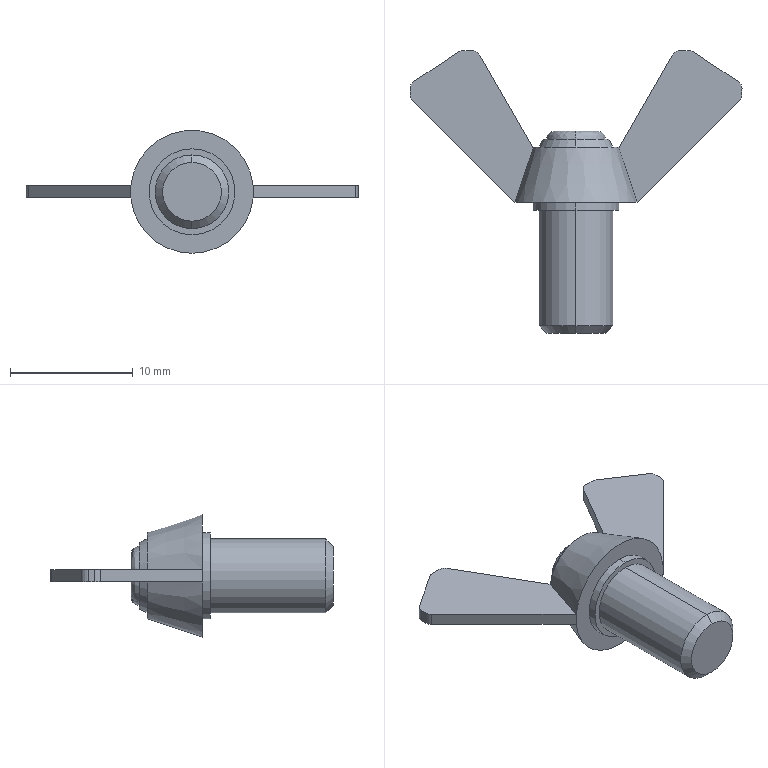Component | SolidWorks | CHOB6-25-3 | 1 solid | 41 faces | volume 711 mm3 | plane 20 | cylinder 12 | cone 7 | spline 2 | commonest cylinder face diameters 1.35 x4 6 x2 7 x2 1.3 x2 1.456 x2